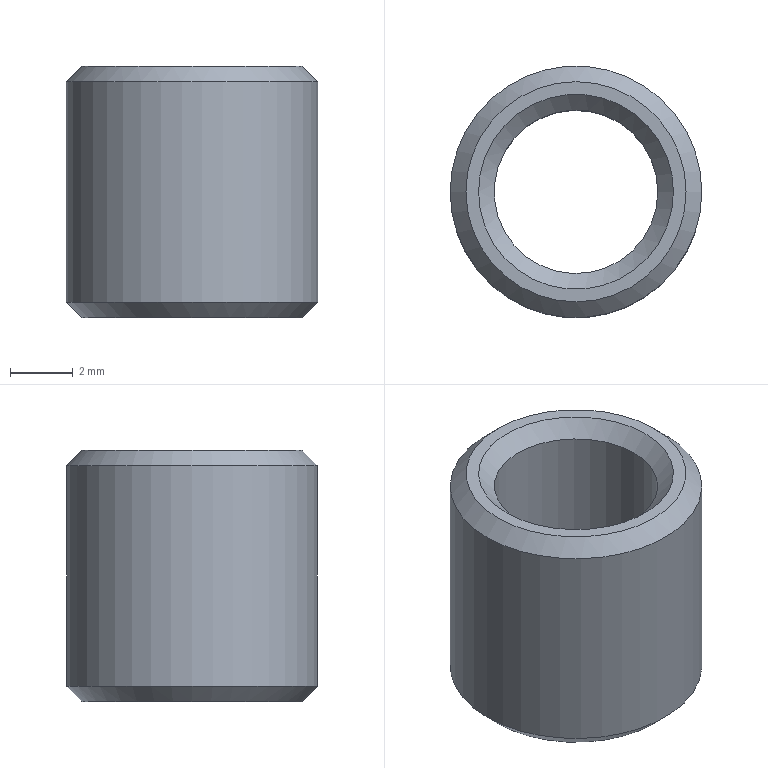Component | NX | ROLLER | 1 solid | 8 faces | box 8 x 8 x 8 mm | volume 222 mm3 | cone 4 | cylinder 2 | plane 2 | commonest cylinder face diameters 8 x1 5.2 x1
STEP:
#1=CARTESIAN_POINT('',(0.,0.,0.));
#2=DIRECTION('',(0.,0.,1.));
#3=DIRECTION('',(1.,0.,0.));
#4=AXIS2_PLACEMENT_3D('',#1,#2,#3);
#5=CARTESIAN_POINT('',(24.453,-0.,-3.5));
#6=VERTEX_POINT('',#5);
#7=CARTESIAN_POINT('',(20.453,-0.,-3.5));
#8=DIRECTION('',(0.,0.,1.));
#9=DIRECTION('',(1.,0.,0.));
#10=AXIS2_PLACEMENT_3D('',#7,#8,#9);
#11=CIRCLE('',#10,4.);
#12=CARTESIAN_POINT('',(20.453,-0.,4.));
#13=DIRECTION('',(0.,0.,-1.));
#14=DIRECTION('',(-1.,0.,0.));
#15=AXIS2_PLACEMENT_3D('',#12,#13,#14);
#16=CYLINDRICAL_SURFACE('',#15,4.);
#17=CARTESIAN_POINT('',(9.425,7.5));
#18=DIRECTION('',(-1.,0.));
#19=VECTOR('',#18,1.);
#20=LINE('',#17,#19);
#21=(GEOMETRIC_REPRESENTATION_CONTEXT(2)PARAMETRIC_REPRESENTATION_CONTEXT()REPRESENTATION_CONTEXT('',''));
#22=DEFINITIONAL_REPRESENTATION('',(#20),#21);
#23=PCURVE('',#16,#22);
#24=CARTESIAN_POINT('',(20.453,-0.,-3.5));
#25=DIRECTION('',(0.,0.,1.));
#26=DIRECTION('',(1.,0.,0.));
#27=AXIS2_PLACEMENT_3D('',#24,#25,#26);
#28=CONICAL_SURFACE('',#27,4.,0.7854);
#29=CARTESIAN_POINT('',(0.,-0.));
#30=DIRECTION('',(1.,0.));
#31=VECTOR('',#30,1.);
#32=LINE('',#29,#31);
#33=(GEOMETRIC_REPRESENTATION_CONTEXT(2)PARAMETRIC_REPRESENTATION_CONTEXT()REPRESENTATION_CONTEXT('',''));
#34=DEFINITIONAL_REPRESENTATION('',(#32),#33);
#35=PCURVE('',#28,#34);
#36=SURFACE_CURVE('',#11,(#23,#35),.PCURVE_S1.);
#37=EDGE_CURVE('',#6,#6,#36,.T.);
#38=ORIENTED_EDGE('',*,*,#37,.T.);
#39=CARTESIAN_POINT('',(24.453,-0.,3.5));
#40=VERTEX_POINT('',#39);
#41=CARTESIAN_POINT('',(24.453,-0.,3.5));
#42=CARTESIAN_POINT('',(24.453,-0.,-3.5));
#43=B_SPLINE_CURVE_WITH_KNOTS('',1,(#41,#42),.UNSPECIFIED.,.F.,.F.,(2,2),(0.5,7.5),.PIECEWISE_BEZIER_KNOTS.);
#44=CARTESIAN_POINT('',(3.142,0.));
#45=DIRECTION('',(0.,1.));
#46=VECTOR('',#45,1.);
#47=LINE('',#44,#46);
#48=(GEOMETRIC_REPRESENTATION_CONTEXT(2)PARAMETRIC_REPRESENTATION_CONTEXT()REPRESENTATION_CONTEXT('',''));
#49=DEFINITIONAL_REPRESENTATION('',(#47),#48);
#50=PCURVE('',#16,#49);
#51=CARTESIAN_POINT('',(9.425,0.));
#52=DIRECTION('',(0.,1.));
#53=VECTOR('',#52,1.);
#54=LINE('',#51,#53);
#55=(GEOMETRIC_REPRESENTATION_CONTEXT(2)PARAMETRIC_REPRESENTATION_CONTEXT()REPRESENTATION_CONTEXT('',''));
#56=DEFINITIONAL_REPRESENTATION('',(#54),#55);
#57=PCURVE('',#16,#56);
#58=SEAM_CURVE('',#43,(#50,#57),.PCURVE_S1.);
#59=EDGE_CURVE('',#40,#6,#58,.T.);
#60=ORIENTED_EDGE('',*,*,#59,.F.);
#61=CARTESIAN_POINT('',(20.453,-0.,3.5));
#62=DIRECTION('',(0.,0.,-1.));
#63=DIRECTION('',(1.,0.,0.));
#64=AXIS2_PLACEMENT_3D('',#61,#62,#63);
#65=CIRCLE('',#64,4.);
#66=CARTESIAN_POINT('',(3.142,0.5));
#67=DIRECTION('',(1.,0.));
#68=VECTOR('',#67,1.);
#69=LINE('',#66,#68);
#70=(GEOMETRIC_REPRESENTATION_CONTEXT(2)PARAMETRIC_REPRESENTATION_CONTEXT()REPRESENTATION_CONTEXT('',''));
#71=DEFINITIONAL_REPRESENTATION('',(#69),#70);
#72=PCURVE('',#16,#71);
#73=CARTESIAN_POINT('',(20.453,-0.,4.));
#74=DIRECTION('',(0.,0.,-1.));
#75=DIRECTION('',(-1.,0.,0.));
#76=AXIS2_PLACEMENT_3D('',#73,#74,#75);
#77=CONICAL_SURFACE('',#76,3.5,0.7854);
#78=CARTESIAN_POINT('',(3.142,0.5));
#79=DIRECTION('',(1.,0.));
#80=VECTOR('',#79,1.);
#81=LINE('',#78,#80);
#82=(GEOMETRIC_REPRESENTATION_CONTEXT(2)PARAMETRIC_REPRESENTATION_CONTEXT()REPRESENTATION_CONTEXT('',''));
#83=DEFINITIONAL_REPRESENTATION('',(#81),#82);
#84=PCURVE('',#77,#83);
#85=SURFACE_CURVE('',#65,(#72,#84),.PCURVE_S1.);
#86=EDGE_CURVE('',#40,#40,#85,.T.);
#87=ORIENTED_EDGE('',*,*,#86,.T.);
#88=ORIENTED_EDGE('',*,*,#59,.T.);
#89=EDGE_LOOP('',(#38,#60,#87,#88));
#90=FACE_BOUND('',#89,.T.);
#91=ADVANCED_FACE('',(#90),#16,.T.);
#92=CARTESIAN_POINT('',(23.053,-0.,-3.5));
#93=VERTEX_POINT('',#92);
#94=CARTESIAN_POINT('',(20.453,-0.,-3.5));
#95=DIRECTION('',(0.,0.,-1.));
#96=DIRECTION('',(1.,0.,0.));
#97=AXIS2_PLACEMENT_3D('',#94,#95,#96);
#98=CIRCLE('',#97,2.6);
#99=CARTESIAN_POINT('',(20.453,-0.,4.));
#100=DIRECTION('',(0.,0.,-1.));
#101=DIRECTION('',(-1.,0.,0.));
#102=AXIS2_PLACEMENT_3D('',#99,#100,#101);
#103=CYLINDRICAL_SURFACE('',#102,2.6);
#104=CARTESIAN_POINT('',(3.142,7.5));
#105=DIRECTION('',(1.,0.));
#106=VECTOR('',#105,1.);
#107=LINE('',#104,#106);
#108=(GEOMETRIC_REPRESENTATION_CONTEXT(2)PARAMETRIC_REPRESENTATION_CONTEXT()REPRESENTATION_CONTEXT('',''));
#109=DEFINITIONAL_REPRESENTATION('',(#107),#108);
#110=PCURVE('',#103,#109);
#111=CARTESIAN_POINT('',(20.453,-0.,-4.));
#112=DIRECTION('',(0.,0.,-1.));
#113=DIRECTION('',(-1.,0.,0.));
#114=AXIS2_PLACEMENT_3D('',#111,#112,#113);
#115=CONICAL_SURFACE('',#114,3.1,0.7854);
#116=CARTESIAN_POINT('',(3.142,-0.5));
#117=DIRECTION('',(1.,0.));
#118=VECTOR('',#117,1.);
#119=LINE('',#116,#118);
#120=(GEOMETRIC_REPRESENTATION_CONTEXT(2)PARAMETRIC_REPRESENTATION_CONTEXT()REPRESENTATION_CONTEXT('',''));
#121=DEFINITIONAL_REPRESENTATION('',(#119),#120);
#122=PCURVE('',#115,#121);
#123=SURFACE_CURVE('',#98,(#110,#122),.PCURVE_S1.);
#124=EDGE_CURVE('',#93,#93,#123,.T.);
#125=ORIENTED_EDGE('',*,*,#124,.F.);
#126=CARTESIAN_POINT('',(23.053,-0.,3.5));
#127=VERTEX_POINT('',#126);
#128=CARTESIAN_POINT('',(23.053,-0.,3.5));
#129=CARTESIAN_POINT('',(23.053,-0.,-3.5));
#130=B_SPLINE_CURVE_WITH_KNOTS('',1,(#128,#129),.UNSPECIFIED.,.F.,.F.,(2,2),(0.5,7.5),.PIECEWISE_BEZIER_KNOTS.);
#131=CARTESIAN_POINT('',(3.142,0.));
#132=DIRECTION('',(0.,1.));
#133=VECTOR('',#132,1.);
#134=LINE('',#131,#133);
#135=(GEOMETRIC_REPRESENTATION_CONTEXT(2)PARAMETRIC_REPRESENTATION_CONTEXT()REPRESENTATION_CONTEXT('',''));
#136=DEFINITIONAL_REPRESENTATION('',(#134),#135);
#137=PCURVE('',#103,#136);
#138=CARTESIAN_POINT('',(9.425,0.));
#139=DIRECTION('',(0.,1.));
#140=VECTOR('',#139,1.);
#141=LINE('',#138,#140);
#142=(GEOMETRIC_REPRESENTATION_CONTEXT(2)PARAMETRIC_REPRESENTATION_CONTEXT()REPRESENTATION_CONTEXT('',''));
#143=DEFINITIONAL_REPRESENTATION('',(#141),#142);
#144=PCURVE('',#103,#143);
#145=SEAM_CURVE('',#130,(#137,#144),.PCURVE_S1.);
#146=EDGE_CURVE('',#127,#93,#145,.T.);
#147=ORIENTED_EDGE('',*,*,#146,.F.);
#148=CARTESIAN_POINT('',(20.453,-0.,3.5));
#149=DIRECTION('',(0.,0.,1.));
#150=DIRECTION('',(1.,0.,0.));
#151=AXIS2_PLACEMENT_3D('',#148,#149,#150);
#152=CIRCLE('',#151,2.6);
#153=CARTESIAN_POINT('',(9.425,0.5));
#154=DIRECTION('',(-1.,0.));
#155=VECTOR('',#154,1.);
#156=LINE('',#153,#155);
#157=(GEOMETRIC_REPRESENTATION_CONTEXT(2)PARAMETRIC_REPRESENTATION_CONTEXT()REPRESENTATION_CONTEXT('',''));
#158=DEFINITIONAL_REPRESENTATION('',(#156),#157);
#159=PCURVE('',#103,#158);
#160=CARTESIAN_POINT('',(20.453,-0.,3.5));
#161=DIRECTION('',(0.,0.,1.));
#162=DIRECTION('',(1.,0.,0.));
#163=AXIS2_PLACEMENT_3D('',#160,#161,#162);
#164=CONICAL_SURFACE('',#163,2.6,0.7854);
#165=CARTESIAN_POINT('',(0.,0.));
#166=DIRECTION('',(1.,0.));
#167=VECTOR('',#166,1.);
#168=LINE('',#165,#167);
#169=(GEOMETRIC_REPRESENTATION_CONTEXT(2)PARAMETRIC_REPRESENTATION_CONTEXT()REPRESENTATION_CONTEXT('',''));
#170=DEFINITIONAL_REPRESENTATION('',(#168),#169);
#171=PCURVE('',#164,#170);
#172=SURFACE_CURVE('',#152,(#159,#171),.PCURVE_S1.);
#173=EDGE_CURVE('',#127,#127,#172,.T.);
#174=ORIENTED_EDGE('',*,*,#173,.F.);
#175=ORIENTED_EDGE('',*,*,#146,.T.);
#176=EDGE_LOOP('',(#125,#147,#174,#175));
#177=FACE_BOUND('',#176,.F.);
#178=ADVANCED_FACE('',(#177),#103,.F.);
#179=CARTESIAN_POINT('',(23.953,-0.,4.));
#180=VERTEX_POINT('',#179);
#181=CARTESIAN_POINT('',(20.453,-0.,4.));
#182=DIRECTION('',(0.,0.,1.));
#183=DIRECTION('',(1.,0.,0.));
#184=AXIS2_PLACEMENT_3D('',#181,#182,#183);
#185=CIRCLE('',#184,3.5);
#186=CARTESIAN_POINT('',(20.453,-0.,4.));
#187=DIRECTION('',(0.,0.,1.));
#188=DIRECTION('',(1.,0.,0.));
#189=AXIS2_PLACEMENT_3D('',#186,#187,#188);
#190=PLANE('',#189);
#191=CARTESIAN_POINT('',(0.,0.));
#192=DIRECTION('',(1.,0.));
#193=AXIS2_PLACEMENT_2D('',#191,#192);
#194=CIRCLE('',#193,3.5);
#195=(GEOMETRIC_REPRESENTATION_CONTEXT(2)PARAMETRIC_REPRESENTATION_CONTEXT()REPRESENTATION_CONTEXT('',''));
#196=DEFINITIONAL_REPRESENTATION('',(#194),#195);
#197=PCURVE('',#190,#196);
#198=CARTESIAN_POINT('',(9.425,-0.));
#199=DIRECTION('',(-1.,0.));
#200=VECTOR('',#199,1.);
#201=LINE('',#198,#200);
#202=(GEOMETRIC_REPRESENTATION_CONTEXT(2)PARAMETRIC_REPRESENTATION_CONTEXT()REPRESENTATION_CONTEXT('',''));
#203=DEFINITIONAL_REPRESENTATION('',(#201),#202);
#204=PCURVE('',#77,#203);
#205=SURFACE_CURVE('',#185,(#197,#204),.PCURVE_S1.);
#206=EDGE_CURVE('',#180,#180,#205,.T.);
#207=ORIENTED_EDGE('',*,*,#206,.T.);
#208=EDGE_LOOP('',(#207));
#209=FACE_BOUND('',#208,.T.);
#210=CARTESIAN_POINT('',(23.553,-0.,4.));
#211=VERTEX_POINT('',#210);
#212=CARTESIAN_POINT('',(20.453,-0.,4.));
#213=DIRECTION('',(0.,0.,-1.));
#214=DIRECTION('',(1.,0.,0.));
#215=AXIS2_PLACEMENT_3D('',#212,#213,#214);
#216=CIRCLE('',#215,3.1);
#217=CARTESIAN_POINT('',(3.1,0.));
#218=CARTESIAN_POINT('',(3.1,-5.369));
#219=CARTESIAN_POINT('',(-1.55,-2.685));
#220=CARTESIAN_POINT('',(-6.2,-0.));
#221=CARTESIAN_POINT('',(-1.55,2.685));
#222=CARTESIAN_POINT('',(3.1,5.369));
#223=CARTESIAN_POINT('',(3.1,0.));
#224=(BOUNDED_CURVE()B_SPLINE_CURVE(2,(#217,#218,#219,#220,#221,#222,#223),.UNSPECIFIED.,.T.,.F.)B_SPLINE_CURVE_WITH_KNOTS((1,2,2,2,2,1),(-2.094,0.,2.094,4.189,6.283,8.378),.UNSPECIFIED.)CURVE()GEOMETRIC_REPRESENTATION_ITEM()RATIONAL_B_SPLINE_CURVE((1.,0.5,1.,0.5,1.,0.5,1.))REPRESENTATION_ITEM(''));
#225=(GEOMETRIC_REPRESENTATION_CONTEXT(2)PARAMETRIC_REPRESENTATION_CONTEXT()REPRESENTATION_CONTEXT('',''));
#226=DEFINITIONAL_REPRESENTATION('',(#224),#225);
#227=PCURVE('',#190,#226);
#228=CARTESIAN_POINT('',(6.283,0.5));
#229=DIRECTION('',(-1.,0.));
#230=VECTOR('',#229,1.);
#231=LINE('',#228,#230);
#232=(GEOMETRIC_REPRESENTATION_CONTEXT(2)PARAMETRIC_REPRESENTATION_CONTEXT()REPRESENTATION_CONTEXT('',''));
#233=DEFINITIONAL_REPRESENTATION('',(#231),#232);
#234=PCURVE('',#164,#233);
#235=SURFACE_CURVE('',#216,(#227,#234),.PCURVE_S1.);
#236=EDGE_CURVE('',#211,#211,#235,.T.);
#237=ORIENTED_EDGE('',*,*,#236,.T.);
#238=EDGE_LOOP('',(#237));
#239=FACE_BOUND('',#238,.T.);
#240=ADVANCED_FACE('',(#209,#239),#190,.T.);
#241=CARTESIAN_POINT('',(23.553,-0.,-4.));
#242=VERTEX_POINT('',#241);
#243=CARTESIAN_POINT('',(20.453,-0.,-4.));
#244=DIRECTION('',(0.,0.,1.));
#245=DIRECTION('',(1.,0.,0.));
#246=AXIS2_PLACEMENT_3D('',#243,#244,#245);
#247=CIRCLE('',#246,3.1);
#248=CARTESIAN_POINT('',(20.453,-0.,-4.));
#249=DIRECTION('',(0.,0.,1.));
#250=DIRECTION('',(1.,0.,0.));
#251=AXIS2_PLACEMENT_3D('',#248,#249,#250);
#252=PLANE('',#251);
#253=CARTESIAN_POINT('',(0.,0.));
#254=DIRECTION('',(1.,0.));
#255=AXIS2_PLACEMENT_2D('',#253,#254);
#256=CIRCLE('',#255,3.1);
#257=(GEOMETRIC_REPRESENTATION_CONTEXT(2)PARAMETRIC_REPRESENTATION_CONTEXT()REPRESENTATION_CONTEXT('',''));
#258=DEFINITIONAL_REPRESENTATION('',(#256),#257);
#259=PCURVE('',#252,#258);
#260=CARTESIAN_POINT('',(9.425,0.));
#261=DIRECTION('',(-1.,0.));
#262=VECTOR('',#261,1.);
#263=LINE('',#260,#262);
#264=(GEOMETRIC_REPRESENTATION_CONTEXT(2)PARAMETRIC_REPRESENTATION_CONTEXT()REPRESENTATION_CONTEXT('',''));
#265=DEFINITIONAL_REPRESENTATION('',(#263),#264);
#266=PCURVE('',#115,#265);
#267=SURFACE_CURVE('',#247,(#259,#266),.PCURVE_S1.);
#268=EDGE_CURVE('',#242,#242,#267,.T.);
#269=ORIENTED_EDGE('',*,*,#268,.T.);
#270=EDGE_LOOP('',(#269));
#271=FACE_BOUND('',#270,.T.);
#272=CARTESIAN_POINT('',(23.953,-0.,-4.));
#273=VERTEX_POINT('',#272);
#274=CARTESIAN_POINT('',(20.453,-0.,-4.));
#275=DIRECTION('',(0.,0.,-1.));
#276=DIRECTION('',(1.,0.,0.));
#277=AXIS2_PLACEMENT_3D('',#274,#275,#276);
#278=CIRCLE('',#277,3.5);
#279=CARTESIAN_POINT('',(3.5,0.));
#280=CARTESIAN_POINT('',(3.5,-6.062));
#281=CARTESIAN_POINT('',(-1.75,-3.031));
#282=CARTESIAN_POINT('',(-7.,-0.));
#283=CARTESIAN_POINT('',(-1.75,3.031));
#284=CARTESIAN_POINT('',(3.5,6.062));
#285=CARTESIAN_POINT('',(3.5,0.));
#286=(BOUNDED_CURVE()B_SPLINE_CURVE(2,(#279,#280,#281,#282,#283,#284,#285),.UNSPECIFIED.,.T.,.F.)B_SPLINE_CURVE_WITH_KNOTS((1,2,2,2,2,1),(-2.094,0.,2.094,4.189,6.283,8.378),.UNSPECIFIED.)CURVE()GEOMETRIC_REPRESENTATION_ITEM()RATIONAL_B_SPLINE_CURVE((1.,0.5,1.,0.5,1.,0.5,1.))REPRESENTATION_ITEM(''));
#287=(GEOMETRIC_REPRESENTATION_CONTEXT(2)PARAMETRIC_REPRESENTATION_CONTEXT()REPRESENTATION_CONTEXT('',''));
#288=DEFINITIONAL_REPRESENTATION('',(#286),#287);
#289=PCURVE('',#252,#288);
#290=CARTESIAN_POINT('',(6.283,-0.5));
#291=DIRECTION('',(-1.,0.));
#292=VECTOR('',#291,1.);
#293=LINE('',#290,#292);
#294=(GEOMETRIC_REPRESENTATION_CONTEXT(2)PARAMETRIC_REPRESENTATION_CONTEXT()REPRESENTATION_CONTEXT('',''));
#295=DEFINITIONAL_REPRESENTATION('',(#293),#294);
#296=PCURVE('',#28,#295);
#297=SURFACE_CURVE('',#278,(#289,#296),.PCURVE_S1.);
#298=EDGE_CURVE('',#273,#273,#297,.T.);
#299=ORIENTED_EDGE('',*,*,#298,.T.);
#300=EDGE_LOOP('',(#299));
#301=FACE_BOUND('',#300,.T.);
#302=ADVANCED_FACE('',(#271,#301),#252,.F.);
#303=ORIENTED_EDGE('',*,*,#124,.T.);
#304=CARTESIAN_POINT('',(23.053,-0.,-3.5));
#305=CARTESIAN_POINT('',(23.553,-0.,-4.));
#306=B_SPLINE_CURVE_WITH_KNOTS('',1,(#304,#305),.UNSPECIFIED.,.F.,.F.,(2,2),(-0.7071,0.),.PIECEWISE_BEZIER_KNOTS.);
#307=CARTESIAN_POINT('',(9.425,0.));
#308=DIRECTION('',(0.,1.));
#309=VECTOR('',#308,1.);
#310=LINE('',#307,#309);
#311=(GEOMETRIC_REPRESENTATION_CONTEXT(2)PARAMETRIC_REPRESENTATION_CONTEXT()REPRESENTATION_CONTEXT('',''));
#312=DEFINITIONAL_REPRESENTATION('',(#310),#311);
#313=PCURVE('',#115,#312);
#314=CARTESIAN_POINT('',(3.142,0.));
#315=DIRECTION('',(0.,1.));
#316=VECTOR('',#315,1.);
#317=LINE('',#314,#316);
#318=(GEOMETRIC_REPRESENTATION_CONTEXT(2)PARAMETRIC_REPRESENTATION_CONTEXT()REPRESENTATION_CONTEXT('',''));
#319=DEFINITIONAL_REPRESENTATION('',(#317),#318);
#320=PCURVE('',#115,#319);
#321=SEAM_CURVE('',#306,(#313,#320),.PCURVE_S1.);
#322=EDGE_CURVE('',#93,#242,#321,.T.);
#323=ORIENTED_EDGE('',*,*,#322,.T.);
#324=ORIENTED_EDGE('',*,*,#268,.T.);
#325=ORIENTED_EDGE('',*,*,#322,.F.);
#326=EDGE_LOOP('',(#303,#323,#324,#325));
#327=FACE_BOUND('',#326,.F.);
#328=ADVANCED_FACE('',(#327),#115,.F.);
#329=ORIENTED_EDGE('',*,*,#298,.F.);
#330=CARTESIAN_POINT('',(23.953,-0.,-4.));
#331=CARTESIAN_POINT('',(24.453,-0.,-3.5));
#332=B_SPLINE_CURVE_WITH_KNOTS('',1,(#330,#331),.UNSPECIFIED.,.F.,.F.,(2,2),(-0.7071,-0.),.PIECEWISE_BEZIER_KNOTS.);
#333=CARTESIAN_POINT('',(6.283,0.));
#334=DIRECTION('',(0.,1.));
#335=VECTOR('',#334,1.);
#336=LINE('',#333,#335);
#337=(GEOMETRIC_REPRESENTATION_CONTEXT(2)PARAMETRIC_REPRESENTATION_CONTEXT()REPRESENTATION_CONTEXT('',''));
#338=DEFINITIONAL_REPRESENTATION('',(#336),#337);
#339=PCURVE('',#28,#338);
#340=CARTESIAN_POINT('',(0.,0.));
#341=DIRECTION('',(0.,1.));
#342=VECTOR('',#341,1.);
#343=LINE('',#340,#342);
#344=(GEOMETRIC_REPRESENTATION_CONTEXT(2)PARAMETRIC_REPRESENTATION_CONTEXT()REPRESENTATION_CONTEXT('',''));
#345=DEFINITIONAL_REPRESENTATION('',(#343),#344);
#346=PCURVE('',#28,#345);
#347=SEAM_CURVE('',#332,(#339,#346),.PCURVE_S1.);
#348=EDGE_CURVE('',#273,#6,#347,.T.);
#349=ORIENTED_EDGE('',*,*,#348,.T.);
#350=ORIENTED_EDGE('',*,*,#37,.F.);
#351=ORIENTED_EDGE('',*,*,#348,.F.);
#352=EDGE_LOOP('',(#329,#349,#350,#351));
#353=FACE_BOUND('',#352,.T.);
#354=ADVANCED_FACE('',(#353),#28,.T.);
#355=ORIENTED_EDGE('',*,*,#86,.F.);
#356=CARTESIAN_POINT('',(23.953,-0.,4.));
#357=CARTESIAN_POINT('',(24.453,-0.,3.5));
#358=B_SPLINE_CURVE_WITH_KNOTS('',1,(#356,#357),.UNSPECIFIED.,.F.,.F.,(2,2),(-0.,0.7071),.PIECEWISE_BEZIER_KNOTS.);
#359=CARTESIAN_POINT('',(3.142,0.));
#360=DIRECTION('',(0.,1.));
#361=VECTOR('',#360,1.);
#362=LINE('',#359,#361);
#363=(GEOMETRIC_REPRESENTATION_CONTEXT(2)PARAMETRIC_REPRESENTATION_CONTEXT()REPRESENTATION_CONTEXT('',''));
#364=DEFINITIONAL_REPRESENTATION('',(#362),#363);
#365=PCURVE('',#77,#364);
#366=CARTESIAN_POINT('',(9.425,0.));
#367=DIRECTION('',(0.,1.));
#368=VECTOR('',#367,1.);
#369=LINE('',#366,#368);
#370=(GEOMETRIC_REPRESENTATION_CONTEXT(2)PARAMETRIC_REPRESENTATION_CONTEXT()REPRESENTATION_CONTEXT('',''));
#371=DEFINITIONAL_REPRESENTATION('',(#369),#370);
#372=PCURVE('',#77,#371);
#373=SEAM_CURVE('',#358,(#365,#372),.PCURVE_S1.);
#374=EDGE_CURVE('',#180,#40,#373,.T.);
#375=ORIENTED_EDGE('',*,*,#374,.F.);
#376=ORIENTED_EDGE('',*,*,#206,.F.);
#377=ORIENTED_EDGE('',*,*,#374,.T.);
#378=EDGE_LOOP('',(#355,#375,#376,#377));
#379=FACE_BOUND('',#378,.T.);
#380=ADVANCED_FACE('',(#379),#77,.T.);
#381=ORIENTED_EDGE('',*,*,#236,.T.);
#382=CARTESIAN_POINT('',(23.053,-0.,3.5));
#383=CARTESIAN_POINT('',(23.553,-0.,4.));
#384=B_SPLINE_CURVE_WITH_KNOTS('',1,(#382,#383),.UNSPECIFIED.,.F.,.F.,(2,2),(0.,0.7071),.PIECEWISE_BEZIER_KNOTS.);
#385=CARTESIAN_POINT('',(0.,0.));
#386=DIRECTION('',(0.,1.));
#387=VECTOR('',#386,1.);
#388=LINE('',#385,#387);
#389=(GEOMETRIC_REPRESENTATION_CONTEXT(2)PARAMETRIC_REPRESENTATION_CONTEXT()REPRESENTATION_CONTEXT('',''));
#390=DEFINITIONAL_REPRESENTATION('',(#388),#389);
#391=PCURVE('',#164,#390);
#392=CARTESIAN_POINT('',(6.283,0.));
#393=DIRECTION('',(0.,1.));
#394=VECTOR('',#393,1.);
#395=LINE('',#392,#394);
#396=(GEOMETRIC_REPRESENTATION_CONTEXT(2)PARAMETRIC_REPRESENTATION_CONTEXT()REPRESENTATION_CONTEXT('',''));
#397=DEFINITIONAL_REPRESENTATION('',(#395),#396);
#398=PCURVE('',#164,#397);
#399=SEAM_CURVE('',#384,(#391,#398),.PCURVE_S1.);
#400=EDGE_CURVE('',#127,#211,#399,.T.);
#401=ORIENTED_EDGE('',*,*,#400,.F.);
#402=ORIENTED_EDGE('',*,*,#173,.T.);
#403=ORIENTED_EDGE('',*,*,#400,.T.);
#404=EDGE_LOOP('',(#381,#401,#402,#403));
#405=FACE_BOUND('',#404,.F.);
#406=ADVANCED_FACE('',(#405),#164,.F.);
#407=CLOSED_SHELL('',(#91,#178,#240,#302,#328,#354,#380,#406));
#408=MANIFOLD_SOLID_BREP('',#407);
#409=(LENGTH_UNIT()NAMED_UNIT(*)SI_UNIT(.MILLI.,.METRE.));
#410=UNCERTAINTY_MEASURE_WITH_UNIT(LENGTH_MEASURE(0.00001),#409,'','');
#411=(NAMED_UNIT(*)PLANE_ANGLE_UNIT()SI_UNIT($,.RADIAN.));
#412=(NAMED_UNIT(*)SI_UNIT($,.STERADIAN.)SOLID_ANGLE_UNIT());
#413=(GEOMETRIC_REPRESENTATION_CONTEXT(3)GLOBAL_UNCERTAINTY_ASSIGNED_CONTEXT((#410))GLOBAL_UNIT_ASSIGNED_CONTEXT((#409,#411,#412))REPRESENTATION_CONTEXT('',''));
#414=ADVANCED_BREP_SHAPE_REPRESENTATION('',(#4,#408),#413);